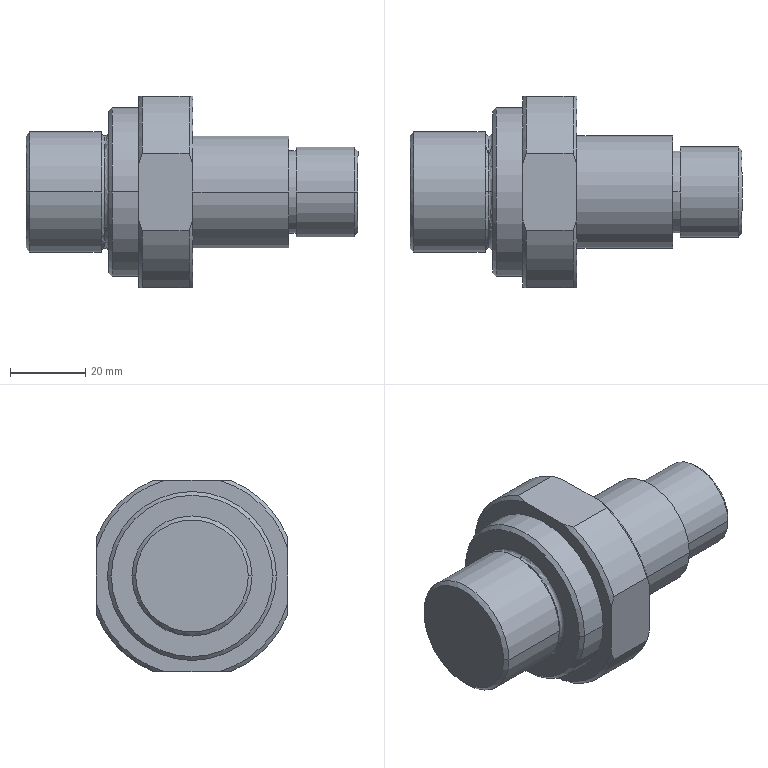Component | SolidWorks | GL9-236--a_b-1 | 1 solid | 43 faces | box 88.5 x 51 x 51 mm | volume 89108 mm3 | cone 14 | cylinder 14 | plane 11 | torus 4 | commonest cylinder face diameters 55 x4 24 x2 22 x2 32 x2 30 x2 45 x2
build123d program:
from build123d import *

# Parameters (mm, degrees)
SKETCH2_R      = 1
SKETCH2_W      = 2
SKETCH2_H      = 1
CHAMFER1_SIZE  = 1
SKETCH3_W      = 30
SKETCH3_H      = 5
SKETCH3_W_2    = 5
SKETCH3_H_2    = 30
EXTRUDE4_DEPTH = 97.668


with BuildPart() as part:
    # Sketch1 → Revolve1 (revolve)
    with BuildSketch(Plane(origin=(0, 0, 0), x_dir=(0, 0, -1), z_dir=(1, 0, 0))):
        Polygon((0, 0), (0, 16), (-22, 16), (-22, 22.5), (-30, 22.5), (-30, 27.5), (-44.5, 27.5), (-44.5, 15), (-70, 15), (-70, 12), (-88.5, 12), (-88.5, 0), align=None)
    revolve(axis=Axis((0, 0, 0), (0, 0, 1)))

    # Sketch2 → Cut-Revolve1 (revolve, cut)
    with BuildSketch(Plane(origin=(0, 0, 0), x_dir=(0, 0, -1), z_dir=(1, 0, 0)), mode=Mode.PRIVATE) as cut_revolve1_sk:
        with Locations((-21, 16)):
            Circle(SKETCH2_R)
        with Locations((-71, 11.5)):
            Rectangle(SKETCH2_W, SKETCH2_H)
    revolve(cut_revolve1_sk.sketch.rotate(Axis((0, 0, 0), (0, 0, 1)), 90), axis=Axis((0, 0, 0), (0, 0, 1)), mode=Mode.SUBTRACT)

    # Chamfer1
    chamfer1_edges = [part.edges().sort_by_distance(p)[0] for p in [
        (0, -27.5, 44.5),
        (0, -27.5, 30),
        (0, -22.5, 22),
        (0, -16, 0),
        (0, -12, 88.5),
    ]]
    chamfer(chamfer1_edges, length=CHAMFER1_SIZE)

    # Sketch3 → Extrude4 (cut, through all)
    with BuildSketch(Plane.XY):
        with Locations((0, 28)):
            Rectangle(SKETCH3_W, SKETCH3_H)
        with Locations((28, 0)):
            Rectangle(SKETCH3_W_2, SKETCH3_H_2)
        with Locations((-28, 0)):
            Rectangle(SKETCH3_W_2, SKETCH3_H_2)
        with Locations((0, -28)):
            Rectangle(SKETCH3_W, SKETCH3_H)
    extrude(amount=EXTRUDE4_DEPTH, mode=Mode.SUBTRACT)


solid = part.part

# Placed as in the assembly
solid = solid.moved(Location((-15, 81, -400), (0, 90, 0)))